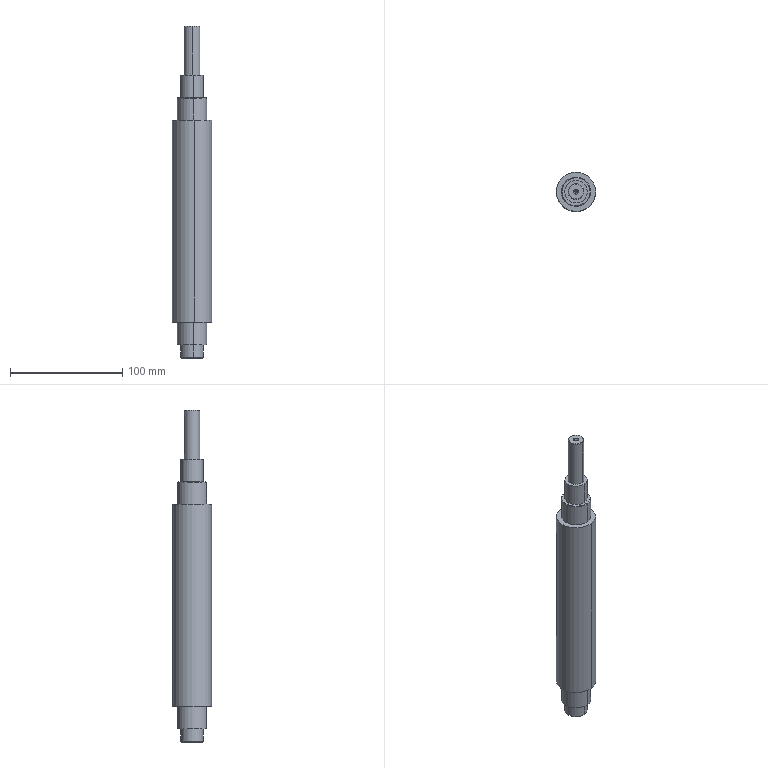Component | SolidWorks | 8TC-A15004-D0-05A-1 | 1 solid | 44 faces | volume 210683 mm3 | cylinder 20 | cone 14 | plane 10 | commonest cylinder face diameters 26 x4 20 x4 2 x4 5 x4 35 x2 14 x2 | material #45